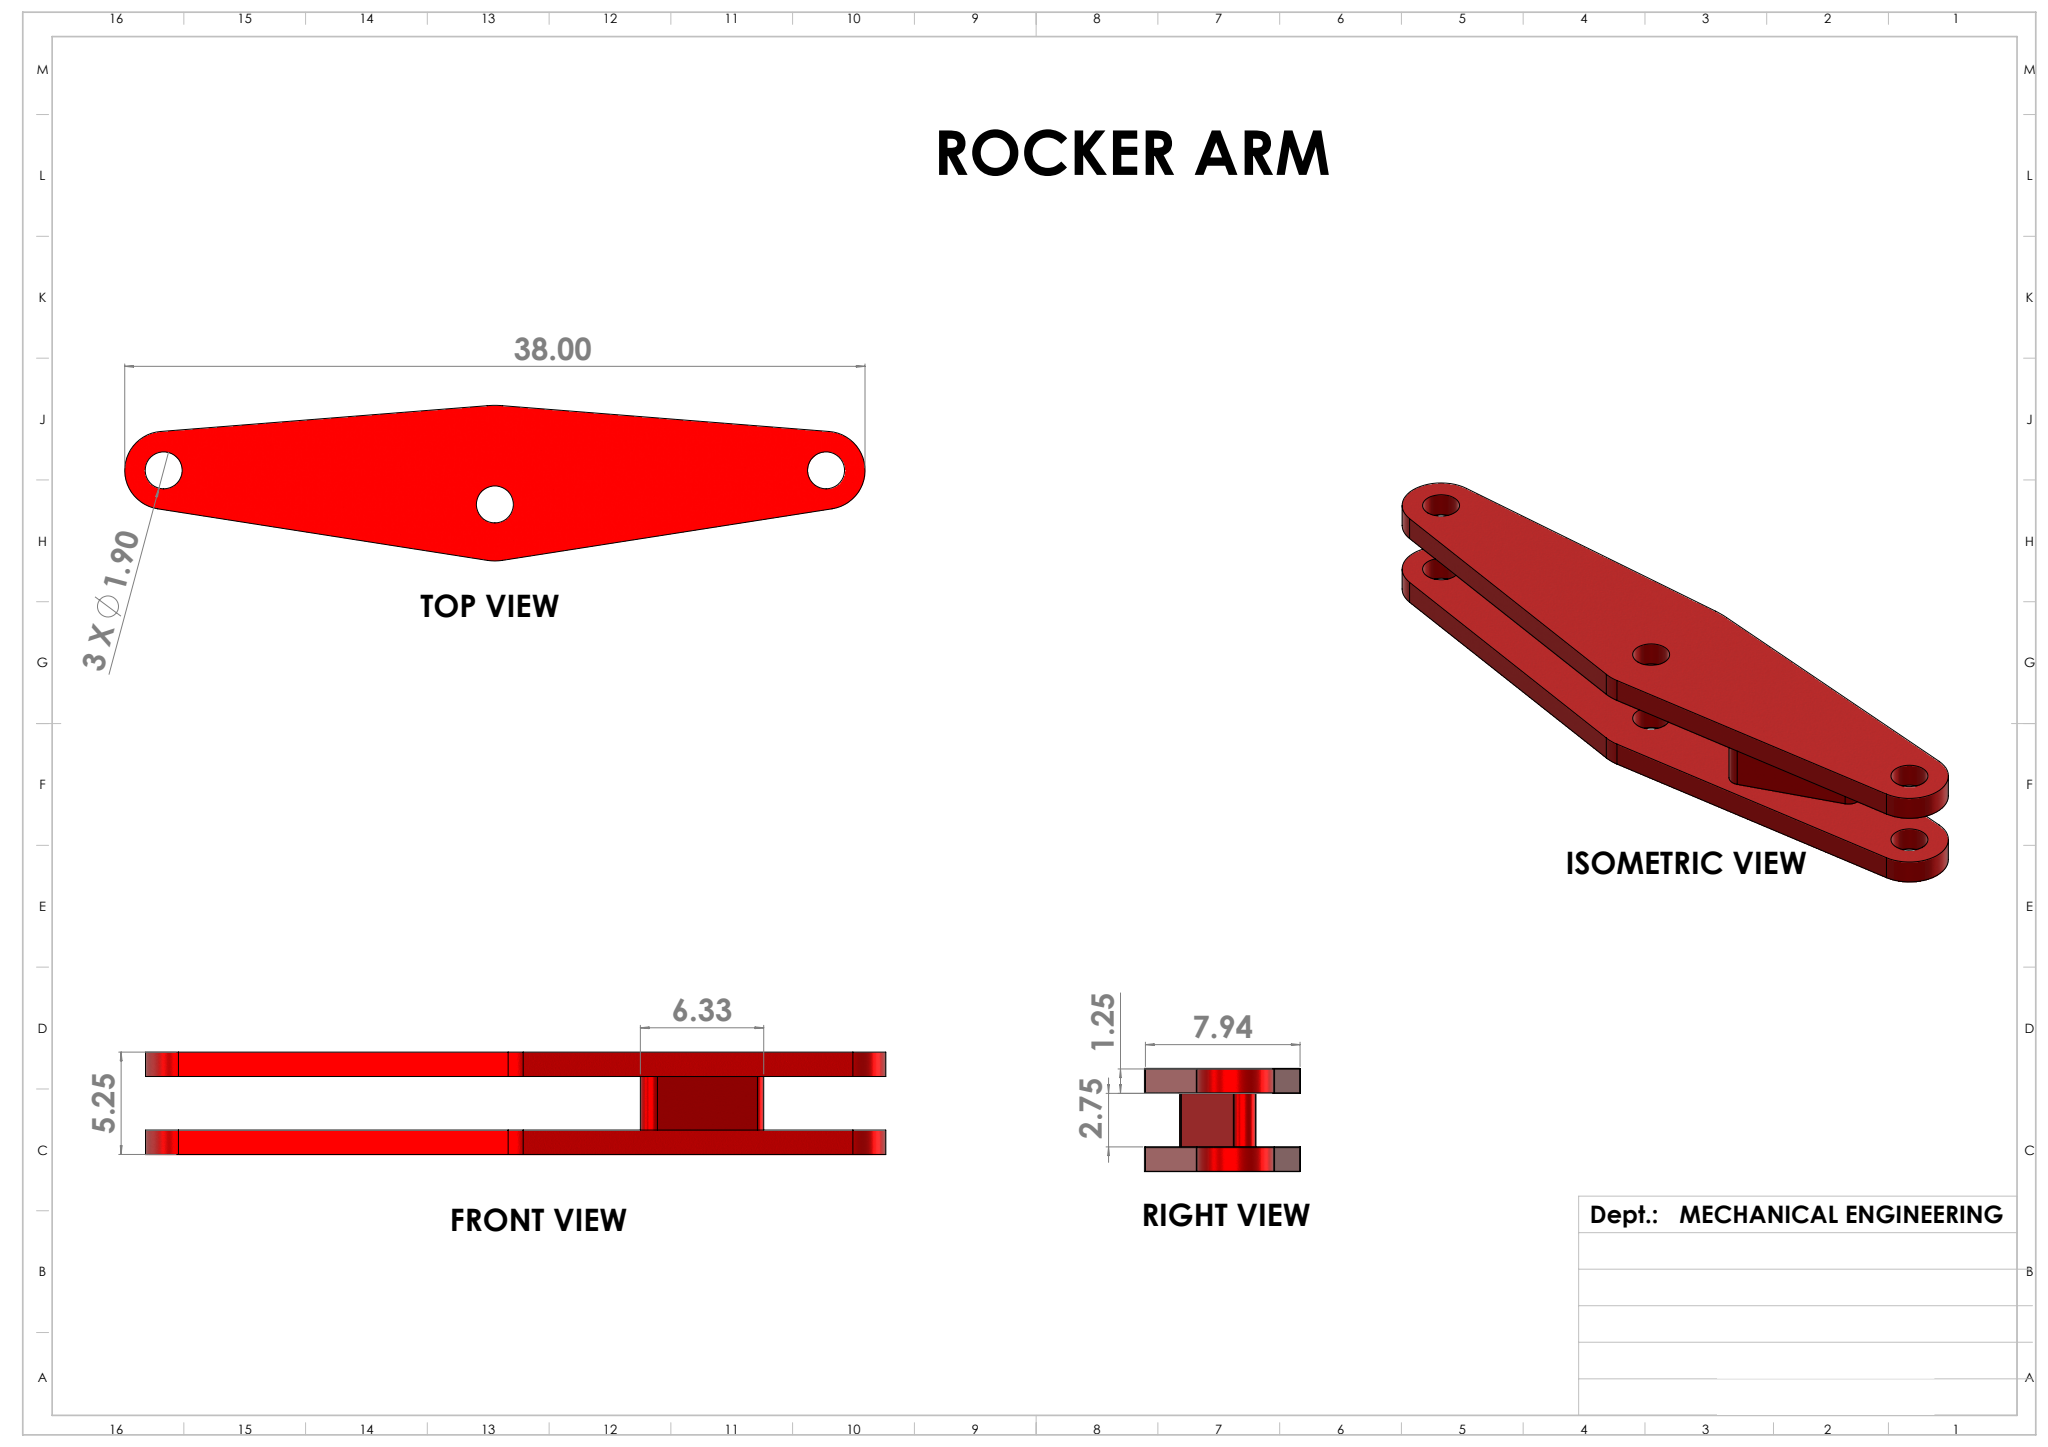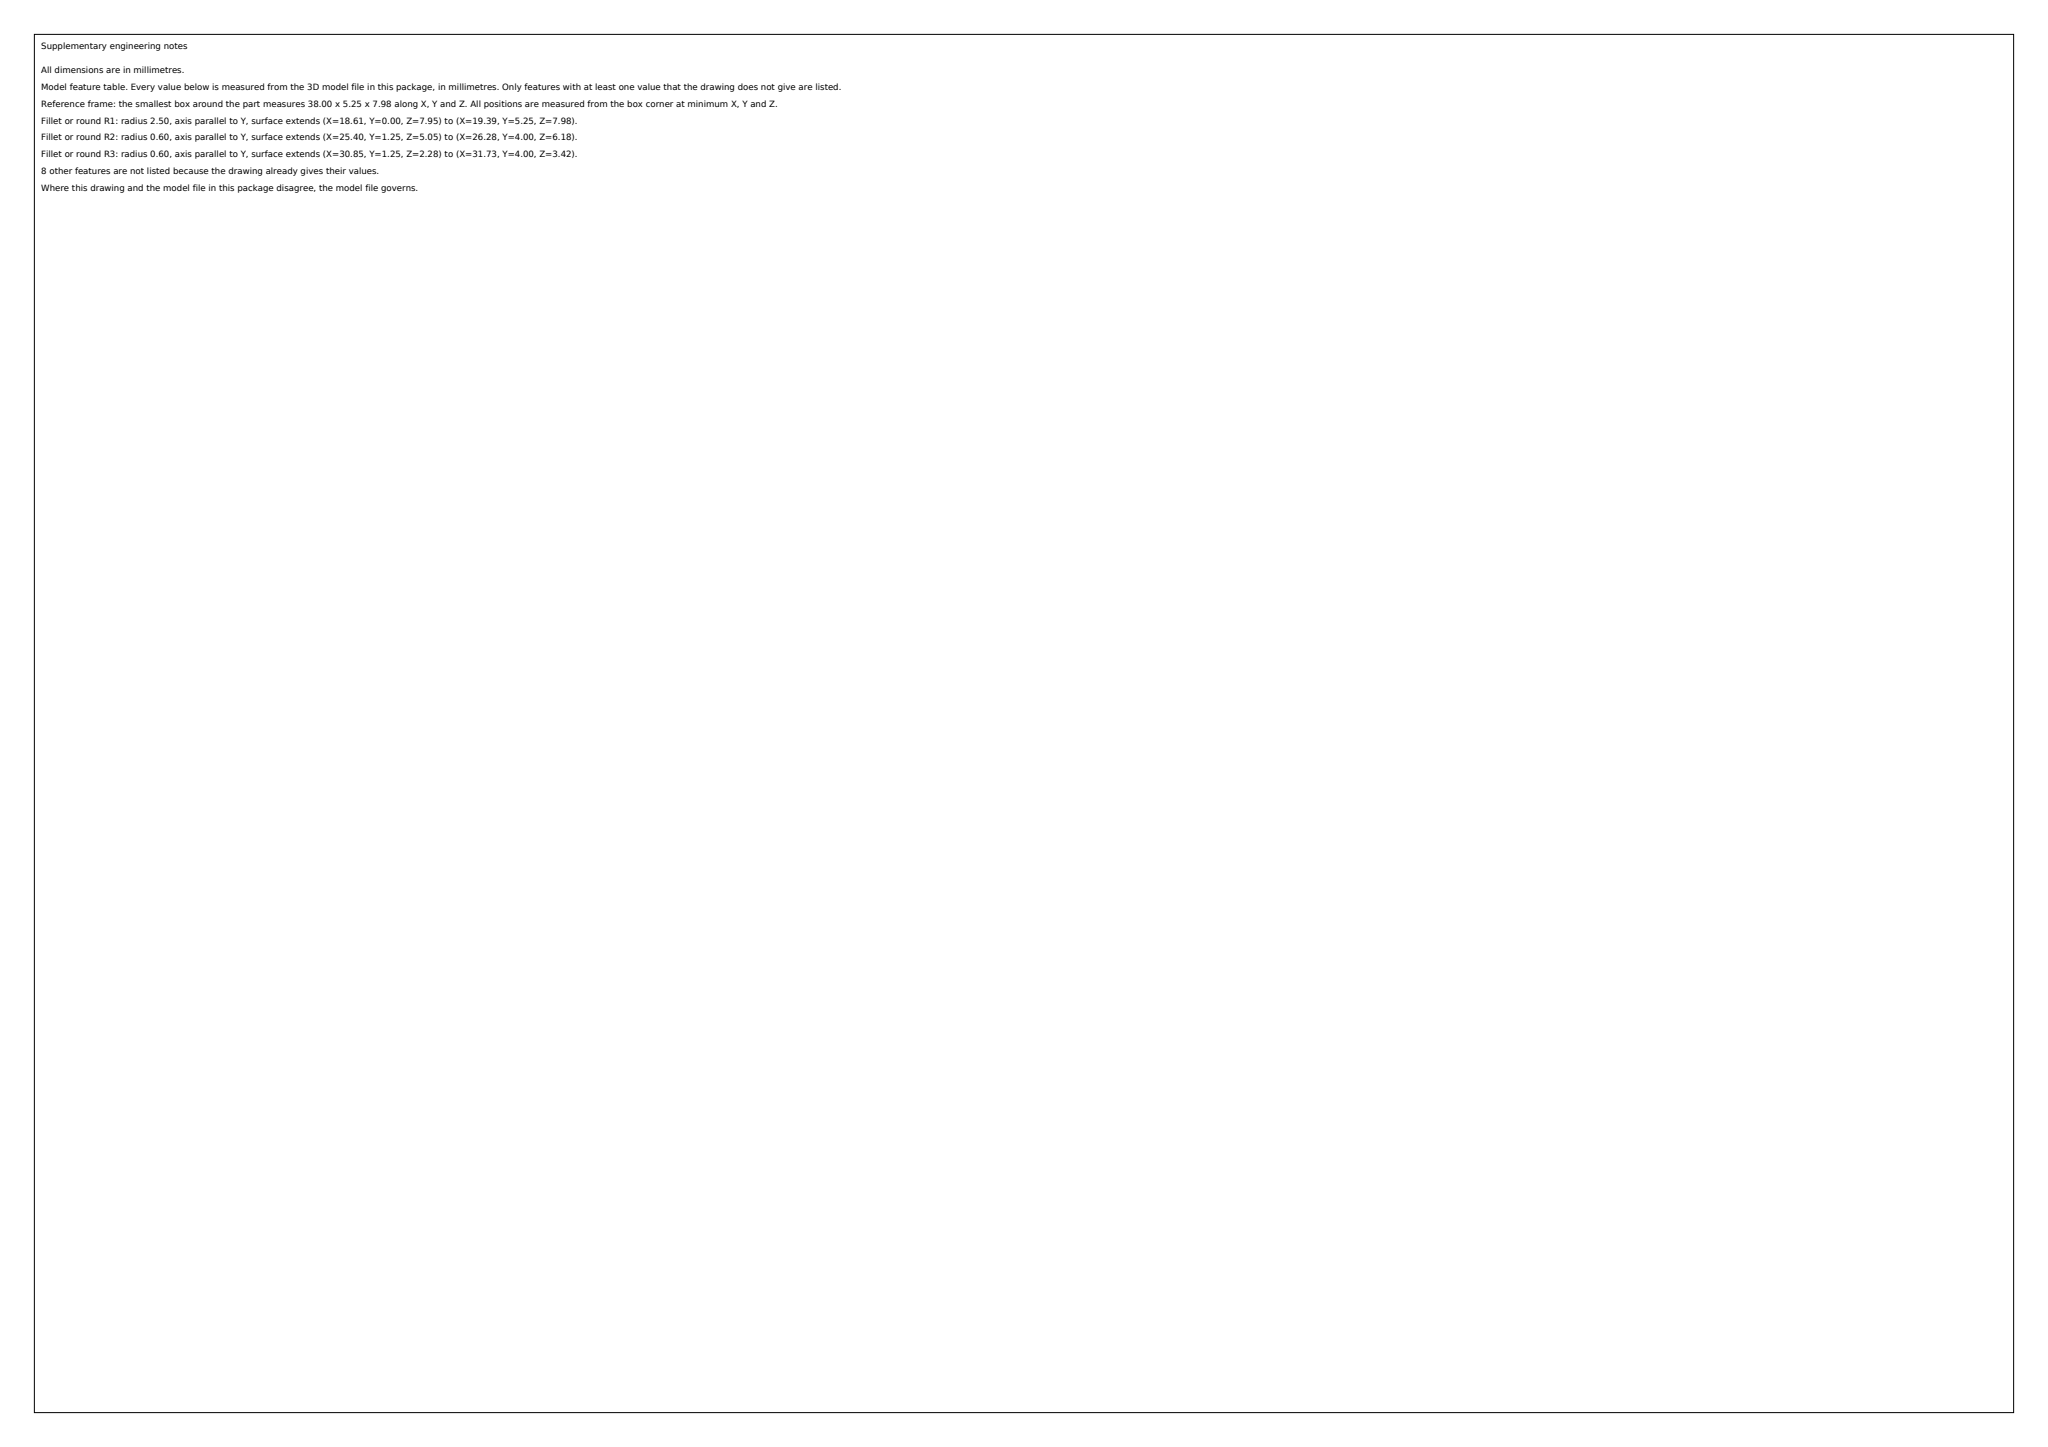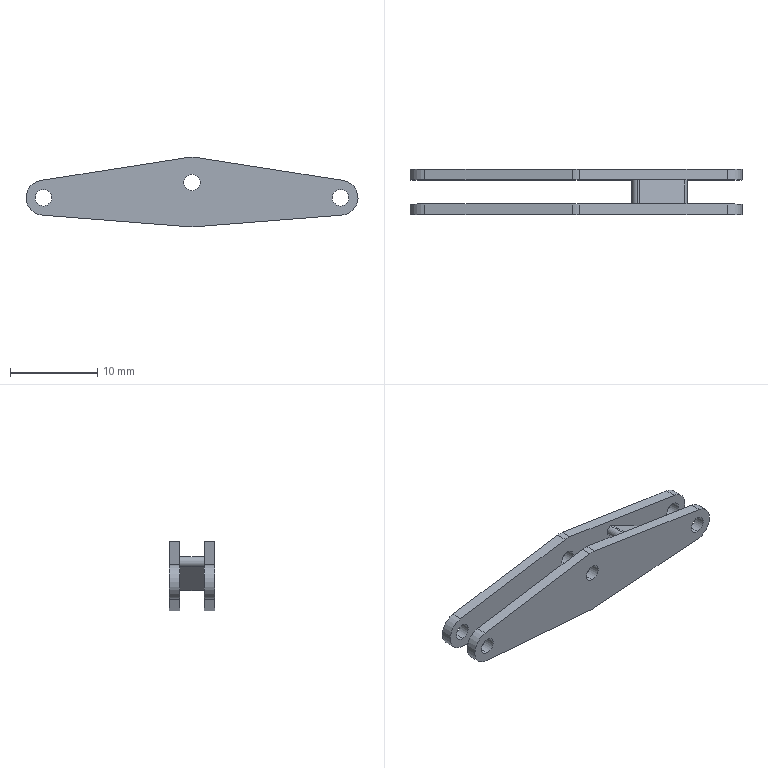Part | SolidWorks | mm | 1 solid | 39 faces | box 38 x 5.25 x 7.98 mm | volume 545 mm3 | cylinder 25 | plane 14 | commonest cylinder face diameters 1.9 x12 10 x4 4 x4 1.2 x3 5 x2
Drawing notes:
SPACER WEB: 1.20 WIDE SLOT-FORM, R0.60 FULL ROUND ENDS, 2.75 LONG BETWEEN ARM FACES (Y=1.25 TO Y=4.00). END-ARC CENTRES AT (X=26.00, Z=5.58) AND (X=31.13, Z=2.88) FROM MIN-CORNER DATUM (X=0 LEFT END FACE, Z=0 BOTTOM EDGE). | from the solid: cylinders dia 1.2 axis y at [26.00,-,5.58] and [31.13,-,2.88], length 2.75; axis planes y=1.25 and y=4.00
TOP-VIEW PROFILE ARCS: R5.00 (Ø10.00) CENTRE AT X=19.00, Z=5.00; R2.50 (Ø5.00) CENTRE AT X=19.00, Z=5.48, BOTH FROM MIN-CORNER DATUM. | from the solid: cylinders dia 10.0 at [19.0,-,5.00] and dia 5.0 at [19.0,-,5.48], axis y
ARM PLATES EACH 1.25 THK; INNER FACES AT Y=1.25 AND Y=4.00, OVERALL WIDTH 5.25 (Y=0 TO Y=5.25). | from the solid: axis_planes y=0.0, 1.25, 4.0, 5.25; bbox_xyz Y=5.25
CENTRE Ø1.90 HOLE AT X=19.00, Z=5.08; END Ø1.90 HOLES AT X=2.00 AND X=36.00, Z=3.33, ALL THRU BOTH ARMS, FROM MIN-CORNER DATUM. | from the solid: cylinders dia 1.9 axis y at [19.0,-,5.08], [2.0,-,3.33], [36.0,-,3.33], length 1.25 each arm
ALL DIMENSIONS IN MILLIMETRES. | from the solid: STEP model units: mm